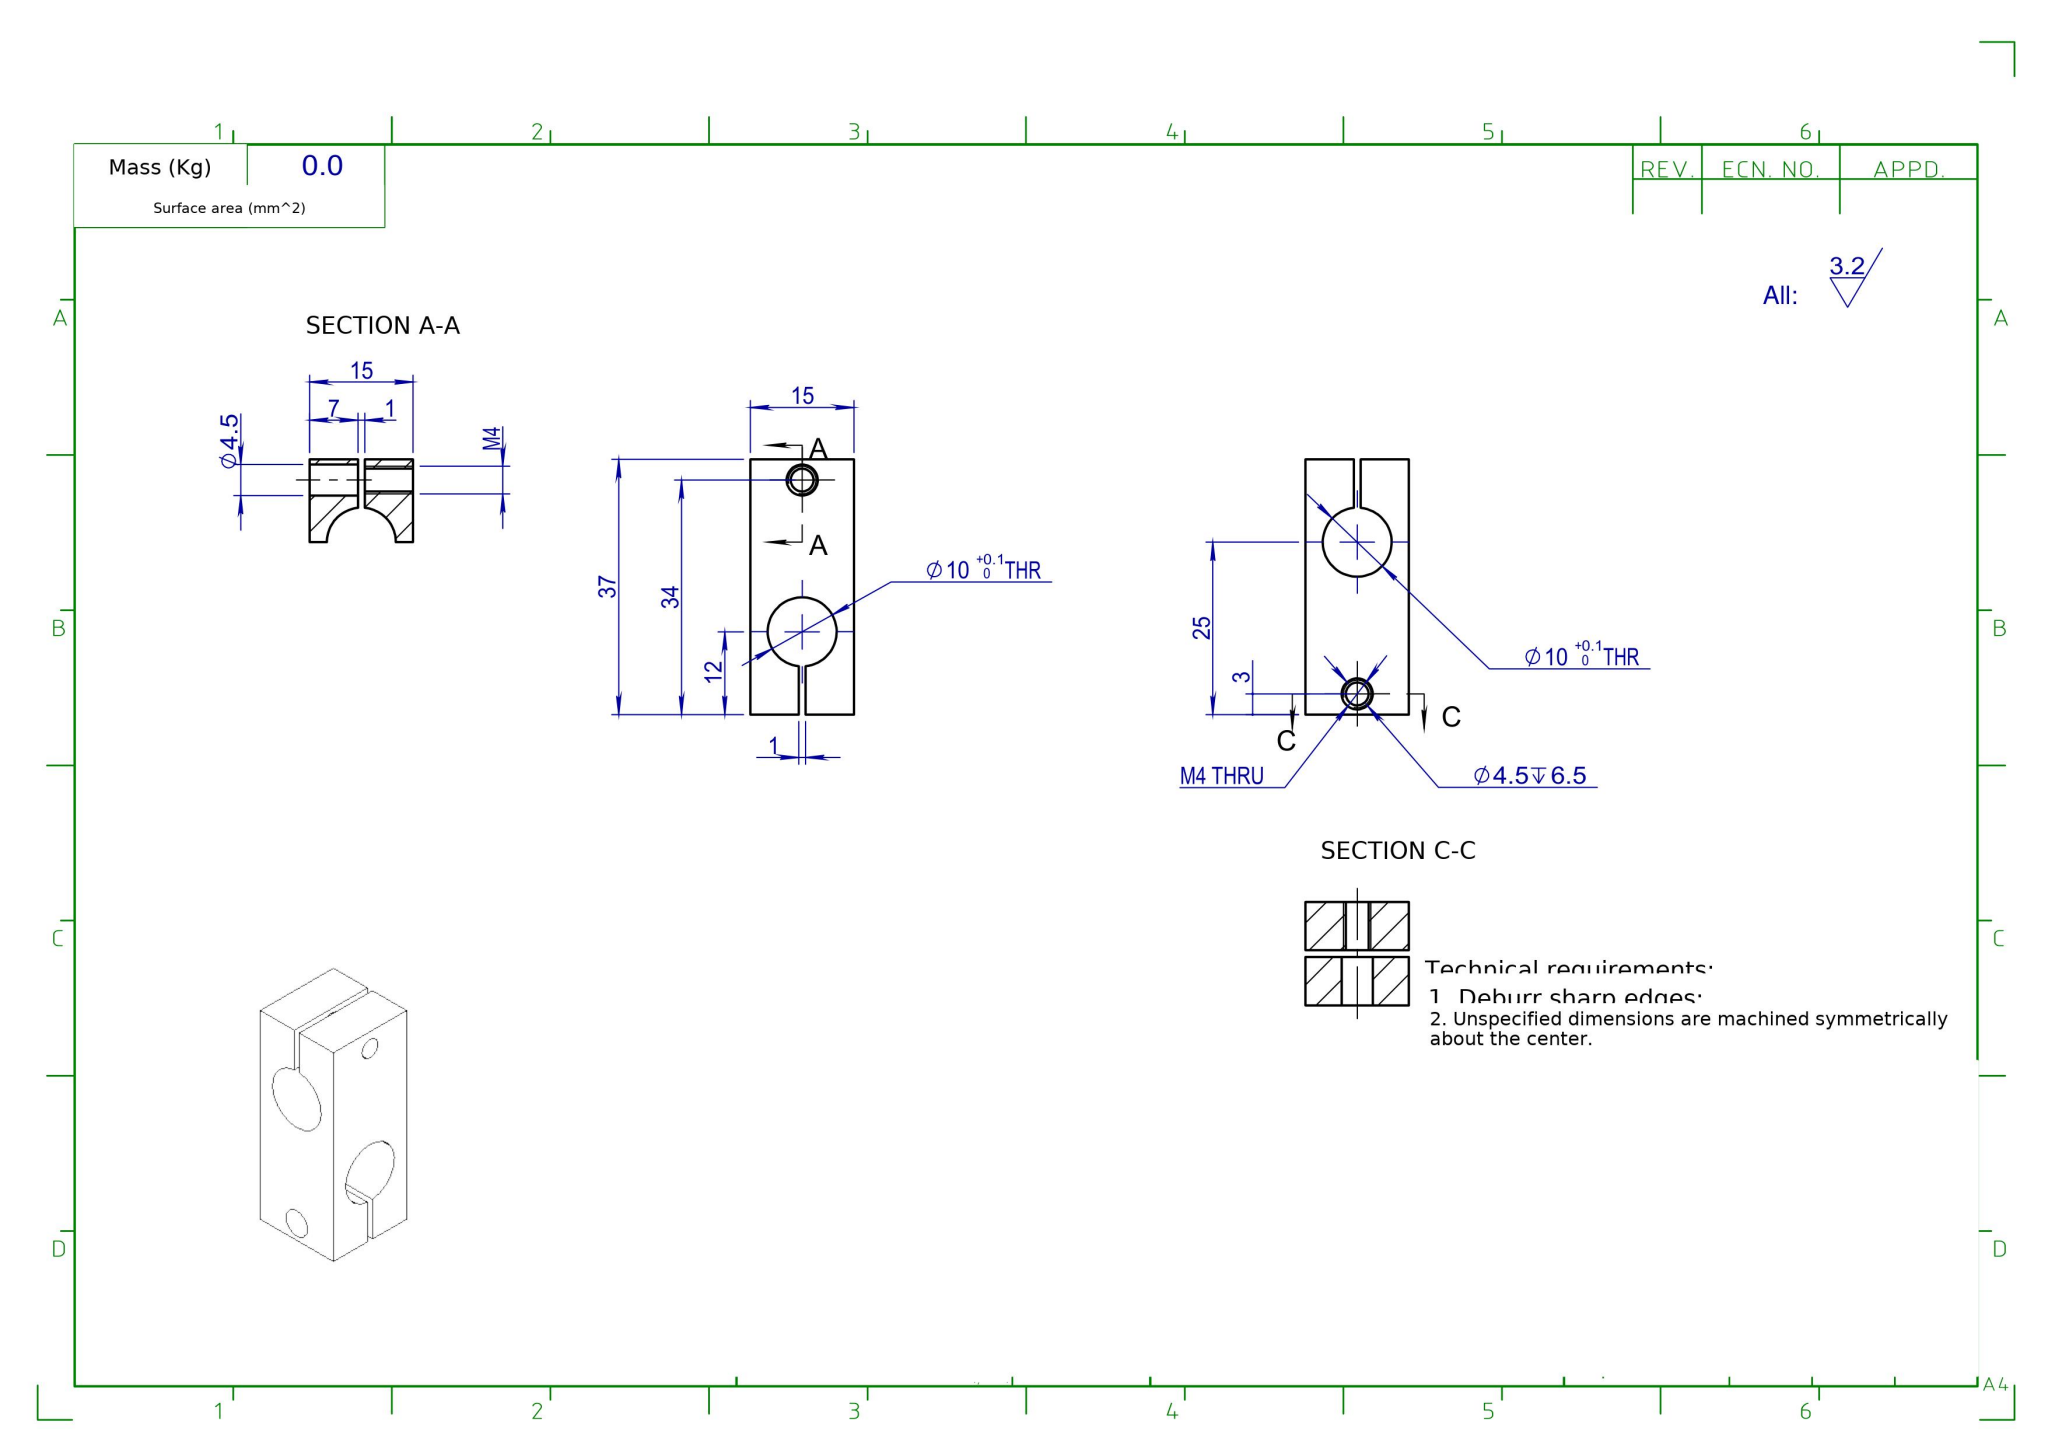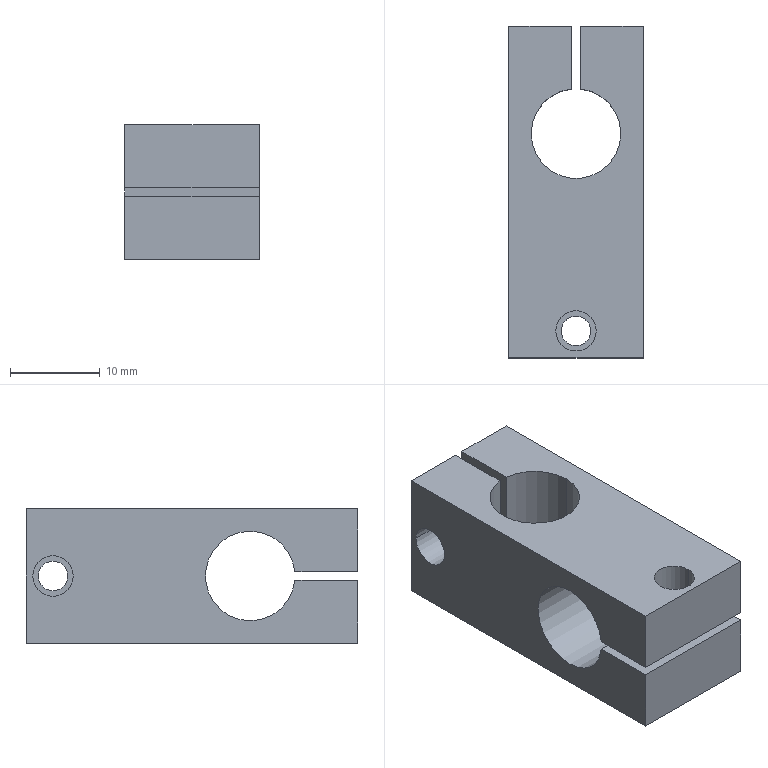Part | SolidWorks | mm | 1 solid | 24 faces | box 15 x 37 x 15 mm | volume 5416 mm3 | cylinder 12 | plane 12 | commonest cylinder face diameters 3.3 x4 4.5 x4 10 x4
build123d program:
from build123d import *

# Parameters (mm, degrees)
SKETCH1_W             = 15
SKETCH1_H             = 37
EXTRUDE1_DEPTH        = 15
SKETCH2_R             = 5
CUT_EXTRUDE1_DEPTH    = 57.588
SKETCH3_R             = 5
CUT_EXTRUDE2_DEPTH    = 57.163
SKETCH4_W             = 1
SKETCH4_H             = 15
CUT_EXTRUDE3_DEPTH    = 57.588
SKETCH5_W             = 1
SKETCH5_H             = 15
CUT_EXTRUDE4_DEPTH    = 57.163
SKETCH6_R             = 2.25
CUT_EXTRUDE5_DEPTH    = 7
SKETCH9_R             = 2.25
CUT_EXTRUDE6_DEPTH    = 7
M4_TAPPED_HOLE2_D     = 3.3
M4_TAPPED_HOLE2_DEPTH = 10.1
M4_TAPPED_HOLE2_TIP   = 0.9914
M4_TAPPED_HOLE3_D     = 3.3


with BuildPart() as part:
    # Sketch1 → Extrude1 (new body)
    with BuildSketch(Plane.XY):
        with Locations((-9.02, -33.503)):
            Rectangle(SKETCH1_W, SKETCH1_H)
    extrude(amount=EXTRUDE1_DEPTH)

    # Sketch2 → Cut-Extrude1 (cut, through all)
    with BuildSketch(Plane.XY.offset(15)):
        with Locations((-9.02, -27.003)):
            Circle(SKETCH2_R)
    extrude(amount=-CUT_EXTRUDE1_DEPTH, mode=Mode.SUBTRACT)

    # Sketch3 → Cut-Extrude2 (cut, through all)
    with BuildSketch(Plane.ZY.offset(16.52)):
        with Locations(Location((7.5, -40.003, 0), (0, 0, 270))):
            Circle(SKETCH3_R)
    extrude(amount=-CUT_EXTRUDE2_DEPTH, mode=Mode.SUBTRACT)

    # Sketch4 → Cut-Extrude3 (cut, through all)
    with BuildSketch(Plane.XY.offset(15)):
        with Locations((-9.02, -22.503)):
            Rectangle(SKETCH4_W, SKETCH4_H)
    extrude(amount=-CUT_EXTRUDE3_DEPTH, mode=Mode.SUBTRACT)

    # Sketch5 → Cut-Extrude4 (cut, through all)
    with BuildSketch(Plane.ZY.offset(16.52)):
        with Locations((7.5, -44.503)):
            Rectangle(SKETCH5_W, SKETCH5_H)
    extrude(amount=-CUT_EXTRUDE4_DEPTH, mode=Mode.SUBTRACT)

    # Sketch6 → Cut-Extrude5 (cut)
    with BuildSketch(Plane.ZY.offset(16.52)):
        with Locations(Location((7.5, -18.003, 0), (0, 0, 270))):
            Circle(SKETCH6_R)
    extrude(amount=-CUT_EXTRUDE5_DEPTH, mode=Mode.SUBTRACT)

    # Sketch9 → Cut-Extrude6 (cut)
    with BuildSketch(Plane.XY.offset(15)):
        with Locations((-9.02, -49.003)):
            Circle(SKETCH9_R)
    extrude(amount=-CUT_EXTRUDE6_DEPTH, mode=Mode.SUBTRACT)

    # M4 Tapped Hole2
    with Locations(Plane.XY.offset(7)):
        with Locations((-9.02, -49.003)):
            Hole(M4_TAPPED_HOLE2_D / 2, depth=M4_TAPPED_HOLE2_DEPTH)
            with Locations((0, 0, -(M4_TAPPED_HOLE2_DEPTH + M4_TAPPED_HOLE2_TIP / 2))):  # 118° drill point
                Cone(0, M4_TAPPED_HOLE2_D / 2, M4_TAPPED_HOLE2_TIP, mode=Mode.SUBTRACT)

    # M4 Tapped Hole3 (through all)
    with Locations(Plane.ZY.offset(8.52)):
        with Locations((7.5, -18.003)):
            Hole(M4_TAPPED_HOLE3_D / 2)


solid = part.part
STEP:
#1=CARTESIAN_POINT('',(-1.52,-18.003,5.85));
#2=VERTEX_POINT('',#1);
#3=CARTESIAN_POINT('',(-1.52,-18.003,9.15));
#4=VERTEX_POINT('',#3);
#5=CARTESIAN_POINT('',(-1.52,-18.003,7.5));
#6=DIRECTION('',(-1.,0.,0.));
#7=DIRECTION('',(0.,0.,1.));
#8=AXIS2_PLACEMENT_3D('',#5,#6,#7);
#9=CIRCLE('',#8,1.65);
#10=EDGE_CURVE('',#2,#4,#9,.T.);
#11=ORIENTED_EDGE('',*,*,#10,.F.);
#12=CARTESIAN_POINT('',(-8.52,-18.003,5.85));
#13=VERTEX_POINT('',#12);
#14=CARTESIAN_POINT('',(-8.52,-18.003,5.85));
#15=DIRECTION('',(-1.,0.,0.));
#16=VECTOR('',#15,1000.);
#17=LINE('',#14,#16);
#18=EDGE_CURVE('',#2,#13,#17,.T.);
#19=ORIENTED_EDGE('',*,*,#18,.T.);
#20=CARTESIAN_POINT('',(-8.52,-18.003,9.15));
#21=VERTEX_POINT('',#20);
#22=CARTESIAN_POINT('',(-8.52,-18.003,7.5));
#23=DIRECTION('',(-1.,0.,0.));
#24=DIRECTION('',(0.,0.,1.));
#25=AXIS2_PLACEMENT_3D('',#22,#23,#24);
#26=CIRCLE('',#25,1.65);
#27=EDGE_CURVE('',#13,#21,#26,.T.);
#28=ORIENTED_EDGE('',*,*,#27,.T.);
#29=CARTESIAN_POINT('',(-8.52,-18.003,9.15));
#30=DIRECTION('',(-1.,0.,0.));
#31=VECTOR('',#30,1000.);
#32=LINE('',#29,#31);
#33=EDGE_CURVE('',#4,#21,#32,.T.);
#34=ORIENTED_EDGE('',*,*,#33,.F.);
#35=EDGE_LOOP('',(#11,#19,#28,#34));
#36=FACE_OUTER_BOUND('',#35,.T.);
#37=CARTESIAN_POINT('',(-8.52,-18.003,7.5));
#38=DIRECTION('',(-1.,0.,0.));
#39=DIRECTION('',(0.,0.,1.));
#40=AXIS2_PLACEMENT_3D('',#37,#38,#39);
#41=CYLINDRICAL_SURFACE('',#40,1.65);
#42=ADVANCED_FACE('',(#36),#41,.F.);
#43=CARTESIAN_POINT('',(-10.67,-49.003,0.));
#44=VERTEX_POINT('',#43);
#45=CARTESIAN_POINT('',(-7.37,-49.003,0.));
#46=VERTEX_POINT('',#45);
#47=CARTESIAN_POINT('',(-9.02,-49.003,0.));
#48=DIRECTION('',(0.,0.,1.));
#49=DIRECTION('',(1.,0.,0.));
#50=AXIS2_PLACEMENT_3D('',#47,#48,#49);
#51=CIRCLE('',#50,1.65);
#52=EDGE_CURVE('',#44,#46,#51,.T.);
#53=ORIENTED_EDGE('',*,*,#52,.F.);
#54=CARTESIAN_POINT('',(-10.67,-49.003,7.));
#55=VERTEX_POINT('',#54);
#56=CARTESIAN_POINT('',(-10.67,-49.003,7.));
#57=DIRECTION('',(0.,0.,1.));
#58=VECTOR('',#57,1000.);
#59=LINE('',#56,#58);
#60=EDGE_CURVE('',#44,#55,#59,.T.);
#61=ORIENTED_EDGE('',*,*,#60,.T.);
#62=CARTESIAN_POINT('',(-7.37,-49.003,7.));
#63=VERTEX_POINT('',#62);
#64=CARTESIAN_POINT('',(-9.02,-49.003,7.));
#65=DIRECTION('',(0.,0.,1.));
#66=DIRECTION('',(1.,0.,0.));
#67=AXIS2_PLACEMENT_3D('',#64,#65,#66);
#68=CIRCLE('',#67,1.65);
#69=EDGE_CURVE('',#55,#63,#68,.T.);
#70=ORIENTED_EDGE('',*,*,#69,.T.);
#71=CARTESIAN_POINT('',(-7.37,-49.003,7.));
#72=DIRECTION('',(0.,0.,1.));
#73=VECTOR('',#72,1000.);
#74=LINE('',#71,#73);
#75=EDGE_CURVE('',#46,#63,#74,.T.);
#76=ORIENTED_EDGE('',*,*,#75,.F.);
#77=EDGE_LOOP('',(#53,#61,#70,#76));
#78=FACE_OUTER_BOUND('',#77,.T.);
#79=CARTESIAN_POINT('',(-9.02,-49.003,7.));
#80=DIRECTION('',(0.,0.,1.));
#81=DIRECTION('',(1.,0.,0.));
#82=AXIS2_PLACEMENT_3D('',#79,#80,#81);
#83=CYLINDRICAL_SURFACE('',#82,1.65);
#84=ADVANCED_FACE('',(#78),#83,.F.);
#85=CARTESIAN_POINT('',(-11.27,-49.003,8.));
#86=VERTEX_POINT('',#85);
#87=CARTESIAN_POINT('',(-6.77,-49.003,8.));
#88=VERTEX_POINT('',#87);
#89=CARTESIAN_POINT('',(-9.02,-49.003,8.));
#90=DIRECTION('',(0.,0.,1.));
#91=DIRECTION('',(1.,0.,0.));
#92=AXIS2_PLACEMENT_3D('',#89,#90,#91);
#93=CIRCLE('',#92,2.25);
#94=EDGE_CURVE('',#86,#88,#93,.T.);
#95=ORIENTED_EDGE('',*,*,#94,.F.);
#96=CARTESIAN_POINT('',(-11.27,-49.003,15.));
#97=VERTEX_POINT('',#96);
#98=CARTESIAN_POINT('',(-11.27,-49.003,8.));
#99=DIRECTION('',(0.,0.,1.));
#100=VECTOR('',#99,1000.);
#101=LINE('',#98,#100);
#102=EDGE_CURVE('',#86,#97,#101,.T.);
#103=ORIENTED_EDGE('',*,*,#102,.T.);
#104=CARTESIAN_POINT('',(-6.77,-49.003,15.));
#105=VERTEX_POINT('',#104);
#106=CARTESIAN_POINT('',(-9.02,-49.003,15.));
#107=DIRECTION('',(0.,0.,1.));
#108=DIRECTION('',(1.,0.,0.));
#109=AXIS2_PLACEMENT_3D('',#106,#107,#108);
#110=CIRCLE('',#109,2.25);
#111=EDGE_CURVE('',#97,#105,#110,.T.);
#112=ORIENTED_EDGE('',*,*,#111,.T.);
#113=CARTESIAN_POINT('',(-6.77,-49.003,8.));
#114=DIRECTION('',(0.,0.,1.));
#115=VECTOR('',#114,1000.);
#116=LINE('',#113,#115);
#117=EDGE_CURVE('',#88,#105,#116,.T.);
#118=ORIENTED_EDGE('',*,*,#117,.F.);
#119=EDGE_LOOP('',(#95,#103,#112,#118));
#120=FACE_OUTER_BOUND('',#119,.T.);
#121=CARTESIAN_POINT('',(-9.02,-49.003,8.));
#122=DIRECTION('',(0.,0.,1.));
#123=DIRECTION('',(1.,0.,0.));
#124=AXIS2_PLACEMENT_3D('',#121,#122,#123);
#125=CYLINDRICAL_SURFACE('',#124,2.25);
#126=ADVANCED_FACE('',(#120),#125,.F.);
#127=CARTESIAN_POINT('',(-9.52,-15.753,7.5));
#128=VERTEX_POINT('',#127);
#129=CARTESIAN_POINT('',(-9.52,-20.253,7.5));
#130=VERTEX_POINT('',#129);
#131=CARTESIAN_POINT('',(-9.52,-18.003,7.5));
#132=DIRECTION('',(-1.,0.,0.));
#133=DIRECTION('',(0.,0.,1.));
#134=AXIS2_PLACEMENT_3D('',#131,#132,#133);
#135=CIRCLE('',#134,2.25);
#136=EDGE_CURVE('',#128,#130,#135,.T.);
#137=ORIENTED_EDGE('',*,*,#136,.F.);
#138=CARTESIAN_POINT('',(-16.52,-15.753,7.5));
#139=VERTEX_POINT('',#138);
#140=CARTESIAN_POINT('',(-8.52,-15.753,7.5));
#141=DIRECTION('',(-1.,-0.,0.));
#142=VECTOR('',#141,1000.);
#143=LINE('',#140,#142);
#144=EDGE_CURVE('',#128,#139,#143,.T.);
#145=ORIENTED_EDGE('',*,*,#144,.T.);
#146=CARTESIAN_POINT('',(-16.52,-20.253,7.5));
#147=VERTEX_POINT('',#146);
#148=CARTESIAN_POINT('',(-16.52,-18.003,7.5));
#149=DIRECTION('',(-1.,-0.,0.));
#150=DIRECTION('',(0.,-1.,0.));
#151=AXIS2_PLACEMENT_3D('',#148,#149,#150);
#152=CIRCLE('',#151,2.25);
#153=EDGE_CURVE('',#139,#147,#152,.T.);
#154=ORIENTED_EDGE('',*,*,#153,.T.);
#155=CARTESIAN_POINT('',(-8.52,-20.253,7.5));
#156=DIRECTION('',(-1.,-0.,0.));
#157=VECTOR('',#156,1000.);
#158=LINE('',#155,#157);
#159=EDGE_CURVE('',#130,#147,#158,.T.);
#160=ORIENTED_EDGE('',*,*,#159,.F.);
#161=EDGE_LOOP('',(#137,#145,#154,#160));
#162=FACE_OUTER_BOUND('',#161,.T.);
#163=CARTESIAN_POINT('',(-8.52,-18.003,7.5));
#164=DIRECTION('',(-1.,-0.,0.));
#165=DIRECTION('',(0.,-1.,0.));
#166=AXIS2_PLACEMENT_3D('',#163,#164,#165);
#167=CYLINDRICAL_SURFACE('',#166,2.25);
#168=ADVANCED_FACE('',(#162),#167,.F.);
#169=CARTESIAN_POINT('',(-14.02,-27.003,0.));
#170=VERTEX_POINT('',#169);
#171=CARTESIAN_POINT('',(-4.02,-27.003,0.));
#172=VERTEX_POINT('',#171);
#173=CARTESIAN_POINT('',(-9.02,-27.003,0.));
#174=DIRECTION('',(0.,0.,1.));
#175=DIRECTION('',(1.,0.,0.));
#176=AXIS2_PLACEMENT_3D('',#173,#174,#175);
#177=CIRCLE('',#176,5.);
#178=EDGE_CURVE('',#170,#172,#177,.T.);
#179=ORIENTED_EDGE('',*,*,#178,.F.);
#180=CARTESIAN_POINT('',(-14.02,-27.003,15.));
#181=VERTEX_POINT('',#180);
#182=CARTESIAN_POINT('',(-14.02,-27.003,0.));
#183=DIRECTION('',(0.,0.,1.));
#184=VECTOR('',#183,1000.);
#185=LINE('',#182,#184);
#186=EDGE_CURVE('',#170,#181,#185,.T.);
#187=ORIENTED_EDGE('',*,*,#186,.T.);
#188=CARTESIAN_POINT('',(-4.02,-27.003,15.));
#189=VERTEX_POINT('',#188);
#190=CARTESIAN_POINT('',(-9.02,-27.003,15.));
#191=DIRECTION('',(0.,0.,1.));
#192=DIRECTION('',(1.,0.,0.));
#193=AXIS2_PLACEMENT_3D('',#190,#191,#192);
#194=CIRCLE('',#193,5.);
#195=EDGE_CURVE('',#181,#189,#194,.T.);
#196=ORIENTED_EDGE('',*,*,#195,.T.);
#197=CARTESIAN_POINT('',(-4.02,-27.003,0.));
#198=DIRECTION('',(0.,0.,1.));
#199=VECTOR('',#198,1000.);
#200=LINE('',#197,#199);
#201=EDGE_CURVE('',#172,#189,#200,.T.);
#202=ORIENTED_EDGE('',*,*,#201,.F.);
#203=EDGE_LOOP('',(#179,#187,#196,#202));
#204=FACE_OUTER_BOUND('',#203,.T.);
#205=CARTESIAN_POINT('',(-9.02,-27.003,0.));
#206=DIRECTION('',(0.,0.,1.));
#207=DIRECTION('',(1.,0.,0.));
#208=AXIS2_PLACEMENT_3D('',#205,#206,#207);
#209=CYLINDRICAL_SURFACE('',#208,5.);
#210=ADVANCED_FACE('',(#204),#209,.F.);
#211=CARTESIAN_POINT('',(-8.52,-22.028,0.));
#212=VERTEX_POINT('',#211);
#213=CARTESIAN_POINT('',(-9.02,-27.003,0.));
#214=DIRECTION('',(0.,0.,1.));
#215=DIRECTION('',(1.,0.,0.));
#216=AXIS2_PLACEMENT_3D('',#213,#214,#215);
#217=CIRCLE('',#216,5.);
#218=EDGE_CURVE('',#172,#212,#217,.T.);
#219=ORIENTED_EDGE('',*,*,#218,.F.);
#220=ORIENTED_EDGE('',*,*,#201,.T.);
#221=CARTESIAN_POINT('',(-8.52,-22.028,15.));
#222=VERTEX_POINT('',#221);
#223=CARTESIAN_POINT('',(-9.02,-27.003,15.));
#224=DIRECTION('',(0.,0.,1.));
#225=DIRECTION('',(1.,0.,0.));
#226=AXIS2_PLACEMENT_3D('',#223,#224,#225);
#227=CIRCLE('',#226,5.);
#228=EDGE_CURVE('',#189,#222,#227,.T.);
#229=ORIENTED_EDGE('',*,*,#228,.T.);
#230=CARTESIAN_POINT('',(-8.52,-22.028,0.));
#231=DIRECTION('',(0.,0.,-1.));
#232=VECTOR('',#231,1000.);
#233=LINE('',#230,#232);
#234=EDGE_CURVE('',#222,#212,#233,.T.);
#235=ORIENTED_EDGE('',*,*,#234,.T.);
#236=EDGE_LOOP('',(#219,#220,#229,#235));
#237=FACE_OUTER_BOUND('',#236,.T.);
#238=CARTESIAN_POINT('',(-9.02,-27.003,0.));
#239=DIRECTION('',(0.,0.,1.));
#240=DIRECTION('',(1.,0.,0.));
#241=AXIS2_PLACEMENT_3D('',#238,#239,#240);
#242=CYLINDRICAL_SURFACE('',#241,5.);
#243=ADVANCED_FACE('',(#237),#242,.F.);
#244=CARTESIAN_POINT('',(-1.52,-52.003,7.));
#245=VERTEX_POINT('',#244);
#246=CARTESIAN_POINT('',(-1.52,-52.003,0.));
#247=VERTEX_POINT('',#246);
#248=CARTESIAN_POINT('',(-1.52,-52.003,15.));
#249=DIRECTION('',(0.,0.,-1.));
#250=VECTOR('',#249,1000.);
#251=LINE('',#248,#250);
#252=EDGE_CURVE('',#245,#247,#251,.T.);
#253=ORIENTED_EDGE('',*,*,#252,.F.);
#254=CARTESIAN_POINT('',(-16.52,-52.003,7.));
#255=VERTEX_POINT('',#254);
#256=CARTESIAN_POINT('',(-1.52,-52.003,7.));
#257=DIRECTION('',(-1.,-0.,0.));
#258=VECTOR('',#257,1000.);
#259=LINE('',#256,#258);
#260=EDGE_CURVE('',#245,#255,#259,.T.);
#261=ORIENTED_EDGE('',*,*,#260,.T.);
#262=CARTESIAN_POINT('',(-16.52,-52.003,0.));
#263=VERTEX_POINT('',#262);
#264=CARTESIAN_POINT('',(-16.52,-52.003,15.));
#265=DIRECTION('',(0.,0.,-1.));
#266=VECTOR('',#265,1000.);
#267=LINE('',#264,#266);
#268=EDGE_CURVE('',#255,#263,#267,.T.);
#269=ORIENTED_EDGE('',*,*,#268,.T.);
#270=CARTESIAN_POINT('',(-16.52,-52.003,0.));
#271=DIRECTION('',(1.,0.,0.));
#272=VECTOR('',#271,1000.);
#273=LINE('',#270,#272);
#274=EDGE_CURVE('',#263,#247,#273,.T.);
#275=ORIENTED_EDGE('',*,*,#274,.T.);
#276=EDGE_LOOP('',(#253,#261,#269,#275));
#277=FACE_OUTER_BOUND('',#276,.T.);
#278=CARTESIAN_POINT('',(-16.52,-52.003,15.));
#279=DIRECTION('',(0.,1.,0.));
#280=DIRECTION('',(0.,0.,1.));
#281=AXIS2_PLACEMENT_3D('',#278,#279,#280);
#282=PLANE('',#281);
#283=ADVANCED_FACE('',(#277),#282,.F.);
#284=CARTESIAN_POINT('',(-1.52,-15.003,0.));
#285=VERTEX_POINT('',#284);
#286=CARTESIAN_POINT('',(-8.52,-15.003,0.));
#287=VERTEX_POINT('',#286);
#288=CARTESIAN_POINT('',(-16.52,-15.003,0.));
#289=DIRECTION('',(-1.,0.,0.));
#290=VECTOR('',#289,1000.);
#291=LINE('',#288,#290);
#292=EDGE_CURVE('',#285,#287,#291,.T.);
#293=ORIENTED_EDGE('',*,*,#292,.T.);
#294=CARTESIAN_POINT('',(-8.52,-15.003,15.));
#295=VERTEX_POINT('',#294);
#296=CARTESIAN_POINT('',(-8.52,-15.003,0.));
#297=DIRECTION('',(0.,0.,1.));
#298=VECTOR('',#297,1000.);
#299=LINE('',#296,#298);
#300=EDGE_CURVE('',#287,#295,#299,.T.);
#301=ORIENTED_EDGE('',*,*,#300,.T.);
#302=CARTESIAN_POINT('',(-1.52,-15.003,15.));
#303=VERTEX_POINT('',#302);
#304=CARTESIAN_POINT('',(-16.52,-15.003,15.));
#305=DIRECTION('',(-1.,0.,0.));
#306=VECTOR('',#305,1000.);
#307=LINE('',#304,#306);
#308=EDGE_CURVE('',#303,#295,#307,.T.);
#309=ORIENTED_EDGE('',*,*,#308,.F.);
#310=CARTESIAN_POINT('',(-1.52,-15.003,15.));
#311=DIRECTION('',(0.,0.,-1.));
#312=VECTOR('',#311,1000.);
#313=LINE('',#310,#312);
#314=EDGE_CURVE('',#303,#285,#313,.T.);
#315=ORIENTED_EDGE('',*,*,#314,.T.);
#316=EDGE_LOOP('',(#293,#301,#309,#315));
#317=FACE_OUTER_BOUND('',#316,.T.);
#318=CARTESIAN_POINT('',(-16.52,-15.003,15.));
#319=DIRECTION('',(0.,-1.,0.));
#320=DIRECTION('',(0.,0.,-1.));
#321=AXIS2_PLACEMENT_3D('',#318,#319,#320);
#322=PLANE('',#321);
#323=ADVANCED_FACE('',(#317),#322,.F.);
#324=CARTESIAN_POINT('',(-16.52,-18.003,7.5));
#325=DIRECTION('',(-1.,-0.,0.));
#326=DIRECTION('',(0.,-1.,0.));
#327=AXIS2_PLACEMENT_3D('',#324,#325,#326);
#328=CIRCLE('',#327,2.25);
#329=EDGE_CURVE('',#147,#139,#328,.T.);
#330=ORIENTED_EDGE('',*,*,#329,.F.);
#331=ORIENTED_EDGE('',*,*,#153,.F.);
#332=EDGE_LOOP('',(#330,#331));
#333=FACE_BOUND('',#332,.T.);
#334=ORIENTED_EDGE('',*,*,#268,.F.);
#335=CARTESIAN_POINT('',(-16.52,-44.978,7.));
#336=VERTEX_POINT('',#335);
#337=CARTESIAN_POINT('',(-16.52,-52.003,7.));
#338=DIRECTION('',(0.,-1.,0.));
#339=VECTOR('',#338,1000.);
#340=LINE('',#337,#339);
#341=EDGE_CURVE('',#336,#255,#340,.T.);
#342=ORIENTED_EDGE('',*,*,#341,.F.);
#343=CARTESIAN_POINT('',(-16.52,-44.978,8.));
#344=VERTEX_POINT('',#343);
#345=CARTESIAN_POINT('',(-16.52,-40.003,7.5));
#346=DIRECTION('',(-1.,-0.,0.));
#347=DIRECTION('',(0.,-1.,0.));
#348=AXIS2_PLACEMENT_3D('',#345,#346,#347);
#349=CIRCLE('',#348,5.);
#350=EDGE_CURVE('',#344,#336,#349,.T.);
#351=ORIENTED_EDGE('',*,*,#350,.F.);
#352=CARTESIAN_POINT('',(-16.52,-52.003,8.));
#353=VERTEX_POINT('',#352);
#354=CARTESIAN_POINT('',(-16.52,-52.003,8.));
#355=DIRECTION('',(-0.,1.,0.));
#356=VECTOR('',#355,1000.);
#357=LINE('',#354,#356);
#358=EDGE_CURVE('',#353,#344,#357,.T.);
#359=ORIENTED_EDGE('',*,*,#358,.F.);
#360=CARTESIAN_POINT('',(-16.52,-52.003,15.));
#361=VERTEX_POINT('',#360);
#362=CARTESIAN_POINT('',(-16.52,-52.003,15.));
#363=DIRECTION('',(0.,0.,-1.));
#364=VECTOR('',#363,1000.);
#365=LINE('',#362,#364);
#366=EDGE_CURVE('',#361,#353,#365,.T.);
#367=ORIENTED_EDGE('',*,*,#366,.F.);
#368=CARTESIAN_POINT('',(-16.52,-15.003,15.));
#369=VERTEX_POINT('',#368);
#370=CARTESIAN_POINT('',(-16.52,-15.003,15.));
#371=DIRECTION('',(0.,-1.,0.));
#372=VECTOR('',#371,1000.);
#373=LINE('',#370,#372);
#374=EDGE_CURVE('',#369,#361,#373,.T.);
#375=ORIENTED_EDGE('',*,*,#374,.F.);
#376=CARTESIAN_POINT('',(-16.52,-15.003,0.));
#377=VERTEX_POINT('',#376);
#378=CARTESIAN_POINT('',(-16.52,-15.003,15.));
#379=DIRECTION('',(0.,0.,-1.));
#380=VECTOR('',#379,1000.);
#381=LINE('',#378,#380);
#382=EDGE_CURVE('',#369,#377,#381,.T.);
#383=ORIENTED_EDGE('',*,*,#382,.T.);
#384=CARTESIAN_POINT('',(-16.52,-15.003,0.));
#385=DIRECTION('',(0.,-1.,0.));
#386=VECTOR('',#385,1000.);
#387=LINE('',#384,#386);
#388=EDGE_CURVE('',#377,#263,#387,.T.);
#389=ORIENTED_EDGE('',*,*,#388,.T.);
#390=EDGE_LOOP('',(#334,#342,#351,#359,#367,#375,#383,#389));
#391=FACE_OUTER_BOUND('',#390,.T.);
#392=CARTESIAN_POINT('',(-16.52,-15.003,15.));
#393=DIRECTION('',(1.,0.,0.));
#394=DIRECTION('',(-0.,1.,0.));
#395=AXIS2_PLACEMENT_3D('',#392,#393,#394);
#396=PLANE('',#395);
#397=ADVANCED_FACE('',(#333,#391),#396,.F.);
#398=ORIENTED_EDGE('',*,*,#366,.T.);
#399=CARTESIAN_POINT('',(-1.52,-52.003,8.));
#400=VERTEX_POINT('',#399);
#401=CARTESIAN_POINT('',(-1.52,-52.003,8.));
#402=DIRECTION('',(-1.,-0.,0.));
#403=VECTOR('',#402,1000.);
#404=LINE('',#401,#403);
#405=EDGE_CURVE('',#400,#353,#404,.T.);
#406=ORIENTED_EDGE('',*,*,#405,.F.);
#407=CARTESIAN_POINT('',(-1.52,-52.003,15.));
#408=VERTEX_POINT('',#407);
#409=CARTESIAN_POINT('',(-1.52,-52.003,15.));
#410=DIRECTION('',(0.,0.,-1.));
#411=VECTOR('',#410,1000.);
#412=LINE('',#409,#411);
#413=EDGE_CURVE('',#408,#400,#412,.T.);
#414=ORIENTED_EDGE('',*,*,#413,.F.);
#415=CARTESIAN_POINT('',(-16.52,-52.003,15.));
#416=DIRECTION('',(1.,0.,0.));
#417=VECTOR('',#416,1000.);
#418=LINE('',#415,#417);
#419=EDGE_CURVE('',#361,#408,#418,.T.);
#420=ORIENTED_EDGE('',*,*,#419,.F.);
#421=EDGE_LOOP('',(#398,#406,#414,#420));
#422=FACE_OUTER_BOUND('',#421,.T.);
#423=CARTESIAN_POINT('',(-16.52,-52.003,15.));
#424=DIRECTION('',(0.,1.,0.));
#425=DIRECTION('',(0.,0.,1.));
#426=AXIS2_PLACEMENT_3D('',#423,#424,#425);
#427=PLANE('',#426);
#428=ADVANCED_FACE('',(#422),#427,.F.);
#429=CARTESIAN_POINT('',(-1.52,-18.003,7.5));
#430=DIRECTION('',(-1.,0.,0.));
#431=DIRECTION('',(0.,0.,1.));
#432=AXIS2_PLACEMENT_3D('',#429,#430,#431);
#433=CIRCLE('',#432,1.65);
#434=EDGE_CURVE('',#4,#2,#433,.T.);
#435=ORIENTED_EDGE('',*,*,#434,.T.);
#436=ORIENTED_EDGE('',*,*,#10,.T.);
#437=EDGE_LOOP('',(#435,#436));
#438=FACE_BOUND('',#437,.T.);
#439=CARTESIAN_POINT('',(-1.52,-44.978,8.));
#440=VERTEX_POINT('',#439);
#441=CARTESIAN_POINT('',(-1.52,-44.978,7.));
#442=VERTEX_POINT('',#441);
#443=CARTESIAN_POINT('',(-1.52,-40.003,7.5));
#444=DIRECTION('',(-1.,-0.,0.));
#445=DIRECTION('',(0.,-1.,0.));
#446=AXIS2_PLACEMENT_3D('',#443,#444,#445);
#447=CIRCLE('',#446,5.);
#448=EDGE_CURVE('',#440,#442,#447,.T.);
#449=ORIENTED_EDGE('',*,*,#448,.T.);
#450=CARTESIAN_POINT('',(-1.52,-52.003,7.));
#451=DIRECTION('',(0.,-1.,0.));
#452=VECTOR('',#451,1000.);
#453=LINE('',#450,#452);
#454=EDGE_CURVE('',#442,#245,#453,.T.);
#455=ORIENTED_EDGE('',*,*,#454,.T.);
#456=ORIENTED_EDGE('',*,*,#252,.T.);
#457=CARTESIAN_POINT('',(-1.52,-15.003,0.));
#458=DIRECTION('',(-0.,1.,0.));
#459=VECTOR('',#458,1000.);
#460=LINE('',#457,#459);
#461=EDGE_CURVE('',#247,#285,#460,.T.);
#462=ORIENTED_EDGE('',*,*,#461,.T.);
#463=ORIENTED_EDGE('',*,*,#314,.F.);
#464=CARTESIAN_POINT('',(-1.52,-15.003,15.));
#465=DIRECTION('',(-0.,1.,0.));
#466=VECTOR('',#465,1000.);
#467=LINE('',#464,#466);
#468=EDGE_CURVE('',#408,#303,#467,.T.);
#469=ORIENTED_EDGE('',*,*,#468,.F.);
#470=ORIENTED_EDGE('',*,*,#413,.T.);
#471=CARTESIAN_POINT('',(-1.52,-52.003,8.));
#472=DIRECTION('',(-0.,1.,0.));
#473=VECTOR('',#472,1000.);
#474=LINE('',#471,#473);
#475=EDGE_CURVE('',#400,#440,#474,.T.);
#476=ORIENTED_EDGE('',*,*,#475,.T.);
#477=EDGE_LOOP('',(#449,#455,#456,#462,#463,#469,#470,#476));
#478=FACE_OUTER_BOUND('',#477,.T.);
#479=CARTESIAN_POINT('',(-1.52,-15.003,15.));
#480=DIRECTION('',(-1.,-0.,0.));
#481=DIRECTION('',(0.,-1.,0.));
#482=AXIS2_PLACEMENT_3D('',#479,#480,#481);
#483=PLANE('',#482);
#484=ADVANCED_FACE('',(#438,#478),#483,.F.);
#485=CARTESIAN_POINT('',(-9.52,-15.003,15.));
#486=VERTEX_POINT('',#485);
#487=CARTESIAN_POINT('',(-16.52,-15.003,15.));
#488=DIRECTION('',(-1.,0.,0.));
#489=VECTOR('',#488,1000.);
#490=LINE('',#487,#489);
#491=EDGE_CURVE('',#486,#369,#490,.T.);
#492=ORIENTED_EDGE('',*,*,#491,.F.);
#493=CARTESIAN_POINT('',(-9.52,-15.003,0.));
#494=VERTEX_POINT('',#493);
#495=CARTESIAN_POINT('',(-9.52,-15.003,0.));
#496=DIRECTION('',(0.,0.,1.));
#497=VECTOR('',#496,1000.);
#498=LINE('',#495,#497);
#499=EDGE_CURVE('',#494,#486,#498,.T.);
#500=ORIENTED_EDGE('',*,*,#499,.F.);
#501=CARTESIAN_POINT('',(-16.52,-15.003,0.));
#502=DIRECTION('',(-1.,0.,0.));
#503=VECTOR('',#502,1000.);
#504=LINE('',#501,#503);
#505=EDGE_CURVE('',#494,#377,#504,.T.);
#506=ORIENTED_EDGE('',*,*,#505,.T.);
#507=ORIENTED_EDGE('',*,*,#382,.F.);
#508=EDGE_LOOP('',(#492,#500,#506,#507));
#509=FACE_OUTER_BOUND('',#508,.T.);
#510=CARTESIAN_POINT('',(-16.52,-15.003,15.));
#511=DIRECTION('',(0.,-1.,0.));
#512=DIRECTION('',(0.,0.,-1.));
#513=AXIS2_PLACEMENT_3D('',#510,#511,#512);
#514=PLANE('',#513);
#515=ADVANCED_FACE('',(#509),#514,.F.);
#516=CARTESIAN_POINT('',(-9.02,-49.003,15.));
#517=DIRECTION('',(0.,0.,1.));
#518=DIRECTION('',(1.,0.,0.));
#519=AXIS2_PLACEMENT_3D('',#516,#517,#518);
#520=CIRCLE('',#519,2.25);
#521=EDGE_CURVE('',#105,#97,#520,.T.);
#522=ORIENTED_EDGE('',*,*,#521,.F.);
#523=ORIENTED_EDGE('',*,*,#111,.F.);
#524=EDGE_LOOP('',(#522,#523));
#525=FACE_BOUND('',#524,.T.);
#526=CARTESIAN_POINT('',(-8.52,-15.003,15.));
#527=DIRECTION('',(-0.,1.,0.));
#528=VECTOR('',#527,1000.);
#529=LINE('',#526,#528);
#530=EDGE_CURVE('',#222,#295,#529,.T.);
#531=ORIENTED_EDGE('',*,*,#530,.F.);
#532=ORIENTED_EDGE('',*,*,#228,.F.);
#533=ORIENTED_EDGE('',*,*,#195,.F.);
#534=CARTESIAN_POINT('',(-9.52,-22.028,15.));
#535=VERTEX_POINT('',#534);
#536=CARTESIAN_POINT('',(-9.02,-27.003,15.));
#537=DIRECTION('',(0.,0.,1.));
#538=DIRECTION('',(1.,0.,0.));
#539=AXIS2_PLACEMENT_3D('',#536,#537,#538);
#540=CIRCLE('',#539,5.);
#541=EDGE_CURVE('',#535,#181,#540,.T.);
#542=ORIENTED_EDGE('',*,*,#541,.F.);
#543=CARTESIAN_POINT('',(-9.52,-15.003,15.));
#544=DIRECTION('',(0.,-1.,0.));
#545=VECTOR('',#544,1000.);
#546=LINE('',#543,#545);
#547=EDGE_CURVE('',#486,#535,#546,.T.);
#548=ORIENTED_EDGE('',*,*,#547,.F.);
#549=ORIENTED_EDGE('',*,*,#491,.T.);
#550=ORIENTED_EDGE('',*,*,#374,.T.);
#551=ORIENTED_EDGE('',*,*,#419,.T.);
#552=ORIENTED_EDGE('',*,*,#468,.T.);
#553=ORIENTED_EDGE('',*,*,#308,.T.);
#554=EDGE_LOOP('',(#531,#532,#533,#542,#548,#549,#550,#551,#552,#553));
#555=FACE_OUTER_BOUND('',#554,.T.);
#556=CARTESIAN_POINT('',(-16.52,-52.003,15.));
#557=DIRECTION('',(0.,0.,1.));
#558=DIRECTION('',(1.,0.,0.));
#559=AXIS2_PLACEMENT_3D('',#556,#557,#558);
#560=PLANE('',#559);
#561=ADVANCED_FACE('',(#525,#555),#560,.T.);
#562=CARTESIAN_POINT('',(-9.02,-49.003,0.));
#563=DIRECTION('',(0.,0.,1.));
#564=DIRECTION('',(1.,0.,0.));
#565=AXIS2_PLACEMENT_3D('',#562,#563,#564);
#566=CIRCLE('',#565,1.65);
#567=EDGE_CURVE('',#46,#44,#566,.T.);
#568=ORIENTED_EDGE('',*,*,#567,.T.);
#569=ORIENTED_EDGE('',*,*,#52,.T.);
#570=EDGE_LOOP('',(#568,#569));
#571=FACE_BOUND('',#570,.T.);
#572=CARTESIAN_POINT('',(-9.52,-22.028,0.));
#573=VERTEX_POINT('',#572);
#574=CARTESIAN_POINT('',(-9.02,-27.003,0.));
#575=DIRECTION('',(0.,0.,1.));
#576=DIRECTION('',(1.,0.,0.));
#577=AXIS2_PLACEMENT_3D('',#574,#575,#576);
#578=CIRCLE('',#577,5.);
#579=EDGE_CURVE('',#573,#170,#578,.T.);
#580=ORIENTED_EDGE('',*,*,#579,.T.);
#581=ORIENTED_EDGE('',*,*,#178,.T.);
#582=ORIENTED_EDGE('',*,*,#218,.T.);
#583=CARTESIAN_POINT('',(-8.52,-15.003,0.));
#584=DIRECTION('',(-0.,1.,0.));
#585=VECTOR('',#584,1000.);
#586=LINE('',#583,#585);
#587=EDGE_CURVE('',#212,#287,#586,.T.);
#588=ORIENTED_EDGE('',*,*,#587,.T.);
#589=ORIENTED_EDGE('',*,*,#292,.F.);
#590=ORIENTED_EDGE('',*,*,#461,.F.);
#591=ORIENTED_EDGE('',*,*,#274,.F.);
#592=ORIENTED_EDGE('',*,*,#388,.F.);
#593=ORIENTED_EDGE('',*,*,#505,.F.);
#594=CARTESIAN_POINT('',(-9.52,-15.003,0.));
#595=DIRECTION('',(0.,-1.,0.));
#596=VECTOR('',#595,1000.);
#597=LINE('',#594,#596);
#598=EDGE_CURVE('',#494,#573,#597,.T.);
#599=ORIENTED_EDGE('',*,*,#598,.T.);
#600=EDGE_LOOP('',(#580,#581,#582,#588,#589,#590,#591,#592,#593,#599));
#601=FACE_OUTER_BOUND('',#600,.T.);
#602=CARTESIAN_POINT('',(-16.52,-52.003,0.));
#603=DIRECTION('',(0.,0.,1.));
#604=DIRECTION('',(1.,0.,0.));
#605=AXIS2_PLACEMENT_3D('',#602,#603,#604);
#606=PLANE('',#605);
#607=ADVANCED_FACE('',(#571,#601),#606,.F.);
#608=ORIENTED_EDGE('',*,*,#186,.F.);
#609=ORIENTED_EDGE('',*,*,#579,.F.);
#610=CARTESIAN_POINT('',(-9.52,-22.028,0.));
#611=DIRECTION('',(0.,0.,1.));
#612=VECTOR('',#611,1000.);
#613=LINE('',#610,#612);
#614=EDGE_CURVE('',#573,#535,#613,.T.);
#615=ORIENTED_EDGE('',*,*,#614,.T.);
#616=ORIENTED_EDGE('',*,*,#541,.T.);
#617=EDGE_LOOP('',(#608,#609,#615,#616));
#618=FACE_OUTER_BOUND('',#617,.T.);
#619=CARTESIAN_POINT('',(-9.02,-27.003,0.));
#620=DIRECTION('',(0.,0.,1.));
#621=DIRECTION('',(1.,0.,0.));
#622=AXIS2_PLACEMENT_3D('',#619,#620,#621);
#623=CYLINDRICAL_SURFACE('',#622,5.);
#624=ADVANCED_FACE('',(#618),#623,.F.);
#625=ORIENTED_EDGE('',*,*,#350,.T.);
#626=CARTESIAN_POINT('',(-1.52,-44.978,7.));
#627=DIRECTION('',(1.,0.,0.));
#628=VECTOR('',#627,1000.);
#629=LINE('',#626,#628);
#630=EDGE_CURVE('',#336,#442,#629,.T.);
#631=ORIENTED_EDGE('',*,*,#630,.T.);
#632=ORIENTED_EDGE('',*,*,#448,.F.);
#633=CARTESIAN_POINT('',(-1.52,-44.978,8.));
#634=DIRECTION('',(-1.,-0.,0.));
#635=VECTOR('',#634,1000.);
#636=LINE('',#633,#635);
#637=EDGE_CURVE('',#440,#344,#636,.T.);
#638=ORIENTED_EDGE('',*,*,#637,.T.);
#639=EDGE_LOOP('',(#625,#631,#632,#638));
#640=FACE_OUTER_BOUND('',#639,.T.);
#641=CARTESIAN_POINT('',(-1.52,-40.003,7.5));
#642=DIRECTION('',(-1.,-0.,0.));
#643=DIRECTION('',(0.,-1.,0.));
#644=AXIS2_PLACEMENT_3D('',#641,#642,#643);
#645=CYLINDRICAL_SURFACE('',#644,5.);
#646=ADVANCED_FACE('',(#640),#645,.F.);
#647=CARTESIAN_POINT('',(-9.52,-18.003,7.5));
#648=DIRECTION('',(-1.,0.,0.));
#649=DIRECTION('',(0.,0.,1.));
#650=AXIS2_PLACEMENT_3D('',#647,#648,#649);
#651=CIRCLE('',#650,2.25);
#652=EDGE_CURVE('',#130,#128,#651,.T.);
#653=ORIENTED_EDGE('',*,*,#652,.T.);
#654=ORIENTED_EDGE('',*,*,#136,.T.);
#655=EDGE_LOOP('',(#653,#654));
#656=FACE_BOUND('',#655,.T.);
#657=ORIENTED_EDGE('',*,*,#598,.F.);
#658=ORIENTED_EDGE('',*,*,#499,.T.);
#659=ORIENTED_EDGE('',*,*,#547,.T.);
#660=ORIENTED_EDGE('',*,*,#614,.F.);
#661=EDGE_LOOP('',(#657,#658,#659,#660));
#662=FACE_OUTER_BOUND('',#661,.T.);
#663=CARTESIAN_POINT('',(-9.52,-15.003,0.));
#664=DIRECTION('',(-1.,0.,0.));
#665=DIRECTION('',(0.,0.,1.));
#666=AXIS2_PLACEMENT_3D('',#663,#664,#665);
#667=PLANE('',#666);
#668=ADVANCED_FACE('',(#656,#662),#667,.F.);
#669=CARTESIAN_POINT('',(-8.52,-18.003,7.5));
#670=DIRECTION('',(-1.,0.,0.));
#671=DIRECTION('',(0.,0.,1.));
#672=AXIS2_PLACEMENT_3D('',#669,#670,#671);
#673=CIRCLE('',#672,1.65);
#674=EDGE_CURVE('',#21,#13,#673,.T.);
#675=ORIENTED_EDGE('',*,*,#674,.F.);
#676=ORIENTED_EDGE('',*,*,#27,.F.);
#677=EDGE_LOOP('',(#675,#676));
#678=FACE_BOUND('',#677,.T.);
#679=ORIENTED_EDGE('',*,*,#530,.T.);
#680=ORIENTED_EDGE('',*,*,#300,.F.);
#681=ORIENTED_EDGE('',*,*,#587,.F.);
#682=ORIENTED_EDGE('',*,*,#234,.F.);
#683=EDGE_LOOP('',(#679,#680,#681,#682));
#684=FACE_OUTER_BOUND('',#683,.T.);
#685=CARTESIAN_POINT('',(-8.52,-15.003,0.));
#686=DIRECTION('',(1.,0.,0.));
#687=DIRECTION('',(-0.,1.,0.));
#688=AXIS2_PLACEMENT_3D('',#685,#686,#687);
#689=PLANE('',#688);
#690=ADVANCED_FACE('',(#678,#684),#689,.F.);
#691=CARTESIAN_POINT('',(-9.02,-49.003,8.));
#692=DIRECTION('',(0.,0.,1.));
#693=DIRECTION('',(1.,0.,0.));
#694=AXIS2_PLACEMENT_3D('',#691,#692,#693);
#695=CIRCLE('',#694,2.25);
#696=EDGE_CURVE('',#88,#86,#695,.T.);
#697=ORIENTED_EDGE('',*,*,#696,.T.);
#698=ORIENTED_EDGE('',*,*,#94,.T.);
#699=EDGE_LOOP('',(#697,#698));
#700=FACE_BOUND('',#699,.T.);
#701=ORIENTED_EDGE('',*,*,#475,.F.);
#702=ORIENTED_EDGE('',*,*,#405,.T.);
#703=ORIENTED_EDGE('',*,*,#358,.T.);
#704=ORIENTED_EDGE('',*,*,#637,.F.);
#705=EDGE_LOOP('',(#701,#702,#703,#704));
#706=FACE_OUTER_BOUND('',#705,.T.);
#707=CARTESIAN_POINT('',(-1.52,-52.003,8.));
#708=DIRECTION('',(0.,0.,1.));
#709=DIRECTION('',(1.,0.,0.));
#710=AXIS2_PLACEMENT_3D('',#707,#708,#709);
#711=PLANE('',#710);
#712=ADVANCED_FACE('',(#700,#706),#711,.F.);
#713=CARTESIAN_POINT('',(-9.02,-49.003,7.));
#714=DIRECTION('',(0.,0.,1.));
#715=DIRECTION('',(1.,0.,0.));
#716=AXIS2_PLACEMENT_3D('',#713,#714,#715);
#717=CIRCLE('',#716,1.65);
#718=EDGE_CURVE('',#63,#55,#717,.T.);
#719=ORIENTED_EDGE('',*,*,#718,.F.);
#720=ORIENTED_EDGE('',*,*,#69,.F.);
#721=EDGE_LOOP('',(#719,#720));
#722=FACE_BOUND('',#721,.T.);
#723=ORIENTED_EDGE('',*,*,#341,.T.);
#724=ORIENTED_EDGE('',*,*,#260,.F.);
#725=ORIENTED_EDGE('',*,*,#454,.F.);
#726=ORIENTED_EDGE('',*,*,#630,.F.);
#727=EDGE_LOOP('',(#723,#724,#725,#726));
#728=FACE_OUTER_BOUND('',#727,.T.);
#729=CARTESIAN_POINT('',(-1.52,-52.003,7.));
#730=DIRECTION('',(0.,0.,-1.));
#731=DIRECTION('',(-1.,0.,0.));
#732=AXIS2_PLACEMENT_3D('',#729,#730,#731);
#733=PLANE('',#732);
#734=ADVANCED_FACE('',(#722,#728),#733,.F.);
#735=ORIENTED_EDGE('',*,*,#144,.F.);
#736=ORIENTED_EDGE('',*,*,#652,.F.);
#737=ORIENTED_EDGE('',*,*,#159,.T.);
#738=ORIENTED_EDGE('',*,*,#329,.T.);
#739=EDGE_LOOP('',(#735,#736,#737,#738));
#740=FACE_OUTER_BOUND('',#739,.T.);
#741=CARTESIAN_POINT('',(-8.52,-18.003,7.5));
#742=DIRECTION('',(-1.,-0.,0.));
#743=DIRECTION('',(0.,-1.,0.));
#744=AXIS2_PLACEMENT_3D('',#741,#742,#743);
#745=CYLINDRICAL_SURFACE('',#744,2.25);
#746=ADVANCED_FACE('',(#740),#745,.F.);
#747=ORIENTED_EDGE('',*,*,#102,.F.);
#748=ORIENTED_EDGE('',*,*,#696,.F.);
#749=ORIENTED_EDGE('',*,*,#117,.T.);
#750=ORIENTED_EDGE('',*,*,#521,.T.);
#751=EDGE_LOOP('',(#747,#748,#749,#750));
#752=FACE_OUTER_BOUND('',#751,.T.);
#753=CARTESIAN_POINT('',(-9.02,-49.003,8.));
#754=DIRECTION('',(0.,0.,1.));
#755=DIRECTION('',(1.,0.,0.));
#756=AXIS2_PLACEMENT_3D('',#753,#754,#755);
#757=CYLINDRICAL_SURFACE('',#756,2.25);
#758=ADVANCED_FACE('',(#752),#757,.F.);
#759=ORIENTED_EDGE('',*,*,#60,.F.);
#760=ORIENTED_EDGE('',*,*,#567,.F.);
#761=ORIENTED_EDGE('',*,*,#75,.T.);
#762=ORIENTED_EDGE('',*,*,#718,.T.);
#763=EDGE_LOOP('',(#759,#760,#761,#762));
#764=FACE_OUTER_BOUND('',#763,.T.);
#765=CARTESIAN_POINT('',(-9.02,-49.003,7.));
#766=DIRECTION('',(0.,0.,1.));
#767=DIRECTION('',(1.,0.,0.));
#768=AXIS2_PLACEMENT_3D('',#765,#766,#767);
#769=CYLINDRICAL_SURFACE('',#768,1.65);
#770=ADVANCED_FACE('',(#764),#769,.F.);
#771=ORIENTED_EDGE('',*,*,#18,.F.);
#772=ORIENTED_EDGE('',*,*,#434,.F.);
#773=ORIENTED_EDGE('',*,*,#33,.T.);
#774=ORIENTED_EDGE('',*,*,#674,.T.);
#775=EDGE_LOOP('',(#771,#772,#773,#774));
#776=FACE_OUTER_BOUND('',#775,.T.);
#777=CARTESIAN_POINT('',(-8.52,-18.003,7.5));
#778=DIRECTION('',(-1.,0.,0.));
#779=DIRECTION('',(0.,0.,1.));
#780=AXIS2_PLACEMENT_3D('',#777,#778,#779);
#781=CYLINDRICAL_SURFACE('',#780,1.65);
#782=ADVANCED_FACE('',(#776),#781,.F.);
#783=CLOSED_SHELL('',(#42,#84,#126,#168,#210,#243,#283,#323,#397,#428,#484,#515,#561,#607,#624,#646,#668,#690,#712,#734,#746,#758,#770,#782));
#784=MANIFOLD_SOLID_BREP('',#783);
#785=CARTESIAN_POINT('',(0.,0.,0.));
#786=DIRECTION('',(0.,0.,1.));
#787=DIRECTION('',(1.,0.,0.));
#788=AXIS2_PLACEMENT_3D('',#785,#786,#787);
#789=(LENGTH_UNIT()NAMED_UNIT(*)SI_UNIT(.MILLI.,.METRE.));
#790=UNCERTAINTY_MEASURE_WITH_UNIT(LENGTH_MEASURE(0.00001),#789,'','');
#791=(NAMED_UNIT(*)PLANE_ANGLE_UNIT()SI_UNIT($,.RADIAN.));
#792=(NAMED_UNIT(*)SI_UNIT($,.STERADIAN.)SOLID_ANGLE_UNIT());
#793=(GEOMETRIC_REPRESENTATION_CONTEXT(3)GLOBAL_UNCERTAINTY_ASSIGNED_CONTEXT((#790))GLOBAL_UNIT_ASSIGNED_CONTEXT((#789,#791,#792))REPRESENTATION_CONTEXT('',''));
#794=ADVANCED_BREP_SHAPE_REPRESENTATION('',(#784,#788),#793);